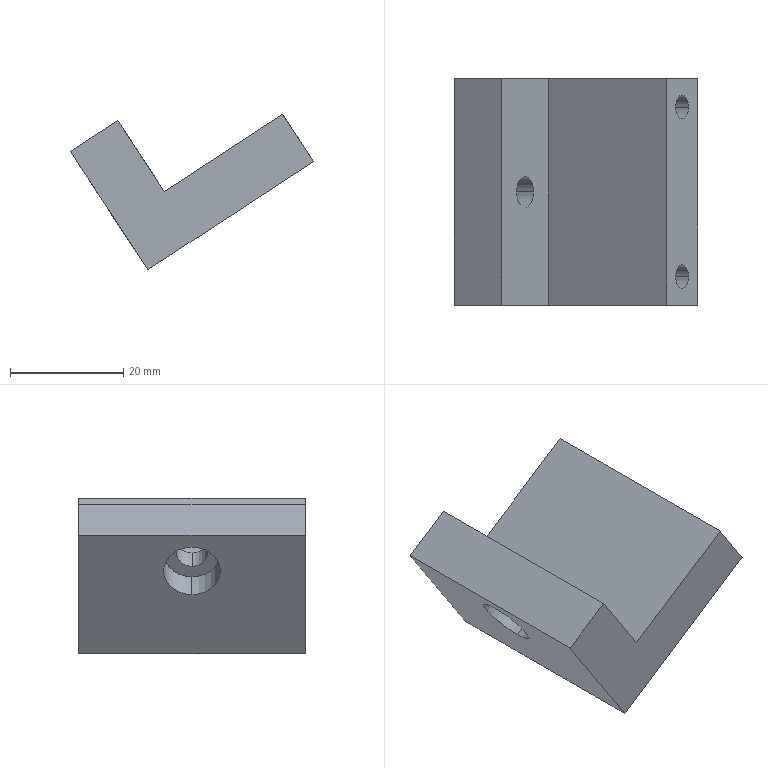Component | SolidWorks | PullSuctionCupMountingPlate-1 | 1 solid | 21 faces | box 42.97 x 40 x 27.52 mm | volume 19095 mm3 | plane 9 | cylinder 8 | cone 4 | commonest cylinder face diameters 4.2 x4 10 x2 5.5 x2
build123d program:
from build123d import *

# Parameters (mm, degrees)
SKETCH1_W                                            = 25
SKETCH1_H                                            = 40
BOSS_EXTRUDE1_DEPTH                                  = 35
SKETCH2_W                                            = 15
SKETCH2_H                                            = 25
CUT_EXTRUDE1_DEPTH                                   = 55.601
M5_TAPPED_HOLE1_D                                    = 4.2
M5_TAPPED_HOLE1_DEPTH                                = 12.4
M5_TAPPED_HOLE1_TIP                                  = 1.262
HOLE_SIZE_ACCORDING_TO_THE_TYPE_OF_HEXAG_D           = 5.5
HOLE_SIZE_ACCORDING_TO_THE_TYPE_OF_HEXAG_CBORE_D     = 10
HOLE_SIZE_ACCORDING_TO_THE_TYPE_OF_HEXAG_CBORE_DEPTH = 5.7


with BuildPart() as part:
    # Sketch1 → Boss-Extrude1 (new body)
    with BuildSketch(Plane.XY):
        Rectangle(SKETCH1_W, SKETCH1_H)
    extrude(amount=BOSS_EXTRUDE1_DEPTH)

    # Sketch2 → Cut-Extrude1 (cut, through all)
    with BuildSketch(Plane(origin=(0, 20, 0), x_dir=(1, 0, 0), z_dir=(0, 1, 0))):
        with Locations((-5, -22.5)):
            Rectangle(SKETCH2_W, SKETCH2_H)
    extrude(amount=-CUT_EXTRUDE1_DEPTH, mode=Mode.SUBTRACT)

    # M5 Tapped Hole1
    with Locations(Plane.XY.offset(35)):
        with Locations((7.5, 15), (7.5, -15)):
            Hole(M5_TAPPED_HOLE1_D / 2, depth=M5_TAPPED_HOLE1_DEPTH)
            with Locations((0, 0, -(M5_TAPPED_HOLE1_DEPTH + M5_TAPPED_HOLE1_TIP / 2))):  # 118° drill point
                Cone(0, M5_TAPPED_HOLE1_D / 2, M5_TAPPED_HOLE1_TIP, mode=Mode.SUBTRACT)

    # Hole Size according to the type of hexag (through all)
    with Locations(Plane(origin=(0, 0, 0), x_dir=(-1, 0, 0), z_dir=(0, 0, -1))):
        with Locations((5, 0)):
            CounterBoreHole(HOLE_SIZE_ACCORDING_TO_THE_TYPE_OF_HEXAG_D / 2, HOLE_SIZE_ACCORDING_TO_THE_TYPE_OF_HEXAG_CBORE_D / 2, HOLE_SIZE_ACCORDING_TO_THE_TYPE_OF_HEXAG_CBORE_DEPTH)


solid = part.part

# Placed as in the assembly
solid = solid.moved(Location((-247.326, -40.454, -152.764), (0, 56.835, 0)))
STEP:
#1=COLOUR_RGB('',0.7922,0.8196,0.9333);
#2=FILL_AREA_STYLE_COLOUR('',#1);
#3=FILL_AREA_STYLE('',(#2));
#4=SURFACE_STYLE_FILL_AREA(#3);
#5=SURFACE_SIDE_STYLE('',(#4));
#6=SURFACE_STYLE_USAGE(.BOTH.,#5);
#7=PRESENTATION_STYLE_ASSIGNMENT((#6));
#8=CARTESIAN_POINT('',(-9.549,-1.593,-5.892));
#9=VERTEX_POINT('',#8);
#10=CARTESIAN_POINT('',(-9.765,-1.593,-5.562));
#11=VERTEX_POINT('',#10);
#12=CARTESIAN_POINT('',(-9.657,-1.593,-5.727));
#13=DIRECTION('',(-0.8371,0.,-0.5471));
#14=DIRECTION('',(-0.5471,-0.,0.8371));
#15=AXIS2_PLACEMENT_3D('',#12,#13,#14);
#16=CIRCLE('',#15,0.1969);
#17=EDGE_CURVE('',#9,#11,#16,.T.);
#18=ORIENTED_EDGE('',*,*,#17,.F.);
#19=CARTESIAN_POINT('',(-9.737,-1.593,-6.014));
#20=VERTEX_POINT('',#19);
#21=CARTESIAN_POINT('',(-9.737,-1.593,-6.014));
#22=DIRECTION('',(-0.8371,0.,-0.5471));
#23=VECTOR('',#22,39.37);
#24=LINE('',#21,#23);
#25=EDGE_CURVE('',#9,#20,#24,.T.);
#26=ORIENTED_EDGE('',*,*,#25,.T.);
#27=CARTESIAN_POINT('',(-9.953,-1.593,-5.685));
#28=VERTEX_POINT('',#27);
#29=CARTESIAN_POINT('',(-9.845,-1.593,-5.85));
#30=DIRECTION('',(-0.8371,0.,-0.5471));
#31=DIRECTION('',(-0.5471,-0.,0.8371));
#32=AXIS2_PLACEMENT_3D('',#29,#30,#31);
#33=CIRCLE('',#32,0.1969);
#34=EDGE_CURVE('',#20,#28,#33,.T.);
#35=ORIENTED_EDGE('',*,*,#34,.T.);
#36=CARTESIAN_POINT('',(-9.953,-1.593,-5.685));
#37=DIRECTION('',(-0.8371,0.,-0.5471));
#38=VECTOR('',#37,39.37);
#39=LINE('',#36,#38);
#40=EDGE_CURVE('',#11,#28,#39,.T.);
#41=ORIENTED_EDGE('',*,*,#40,.F.);
#42=EDGE_LOOP('',(#18,#26,#35,#41));
#43=FACE_OUTER_BOUND('',#42,.T.);
#44=CARTESIAN_POINT('',(-9.845,-1.593,-5.85));
#45=DIRECTION('',(-0.8371,0.,-0.5471));
#46=DIRECTION('',(-0.5471,-0.,0.8371));
#47=AXIS2_PLACEMENT_3D('',#44,#45,#46);
#48=CYLINDRICAL_SURFACE('',#47,0.1969);
#49=ADVANCED_FACE('',(#43),#48,.F.);
#50=CARTESIAN_POINT('',(-9.456,-1.593,-5.725));
#51=VERTEX_POINT('',#50);
#52=CARTESIAN_POINT('',(-9.575,-1.593,-5.544));
#53=VERTEX_POINT('',#52);
#54=CARTESIAN_POINT('',(-9.515,-1.593,-5.634));
#55=DIRECTION('',(-0.8371,0.,-0.5471));
#56=DIRECTION('',(-0.5471,-0.,0.8371));
#57=AXIS2_PLACEMENT_3D('',#54,#55,#56);
#58=CIRCLE('',#57,0.1083);
#59=EDGE_CURVE('',#51,#53,#58,.T.);
#60=ORIENTED_EDGE('',*,*,#59,.F.);
#61=CARTESIAN_POINT('',(-9.598,-1.593,-5.817));
#62=VERTEX_POINT('',#61);
#63=CARTESIAN_POINT('',(-9.786,-1.593,-5.94));
#64=DIRECTION('',(-0.8371,0.,-0.5471));
#65=VECTOR('',#64,39.37);
#66=LINE('',#63,#65);
#67=EDGE_CURVE('',#51,#62,#66,.T.);
#68=ORIENTED_EDGE('',*,*,#67,.T.);
#69=CARTESIAN_POINT('',(-9.716,-1.593,-5.636));
#70=VERTEX_POINT('',#69);
#71=CARTESIAN_POINT('',(-9.657,-1.593,-5.727));
#72=DIRECTION('',(-0.8371,0.,-0.5471));
#73=DIRECTION('',(-0.5471,-0.,0.8371));
#74=AXIS2_PLACEMENT_3D('',#71,#72,#73);
#75=CIRCLE('',#74,0.1083);
#76=EDGE_CURVE('',#62,#70,#75,.T.);
#77=ORIENTED_EDGE('',*,*,#76,.T.);
#78=CARTESIAN_POINT('',(-9.904,-1.593,-5.759));
#79=DIRECTION('',(-0.8371,0.,-0.5471));
#80=VECTOR('',#79,39.37);
#81=LINE('',#78,#80);
#82=EDGE_CURVE('',#53,#70,#81,.T.);
#83=ORIENTED_EDGE('',*,*,#82,.F.);
#84=EDGE_LOOP('',(#60,#68,#77,#83));
#85=FACE_OUTER_BOUND('',#84,.T.);
#86=CARTESIAN_POINT('',(-9.845,-1.593,-5.85));
#87=DIRECTION('',(-0.8371,0.,-0.5471));
#88=DIRECTION('',(-0.5471,-0.,0.8371));
#89=AXIS2_PLACEMENT_3D('',#86,#87,#88);
#90=CYLINDRICAL_SURFACE('',#89,0.1083);
#91=ADVANCED_FACE('',(#85),#90,.F.);
#92=CARTESIAN_POINT('',(-8.876,-1.002,-5.706));
#93=VERTEX_POINT('',#92);
#94=CARTESIAN_POINT('',(-8.786,-1.002,-5.844));
#95=VERTEX_POINT('',#94);
#96=CARTESIAN_POINT('',(-8.831,-1.002,-5.775));
#97=DIRECTION('',(0.8371,-0.,0.5471));
#98=DIRECTION('',(0.5471,0.,-0.8371));
#99=AXIS2_PLACEMENT_3D('',#96,#97,#98);
#100=CIRCLE('',#99,0.08268);
#101=EDGE_CURVE('',#93,#95,#100,.T.);
#102=ORIENTED_EDGE('',*,*,#101,.F.);
#103=CARTESIAN_POINT('',(-8.467,-1.002,-5.438));
#104=VERTEX_POINT('',#103);
#105=CARTESIAN_POINT('',(-8.467,-1.002,-5.438));
#106=DIRECTION('',(0.8371,-0.,0.5471));
#107=VECTOR('',#106,39.37);
#108=LINE('',#105,#107);
#109=EDGE_CURVE('',#93,#104,#108,.T.);
#110=ORIENTED_EDGE('',*,*,#109,.T.);
#111=CARTESIAN_POINT('',(-8.377,-1.002,-5.577));
#112=VERTEX_POINT('',#111);
#113=CARTESIAN_POINT('',(-8.422,-1.002,-5.508));
#114=DIRECTION('',(0.8371,-0.,0.5471));
#115=DIRECTION('',(0.5471,0.,-0.8371));
#116=AXIS2_PLACEMENT_3D('',#113,#114,#115);
#117=CIRCLE('',#116,0.08268);
#118=EDGE_CURVE('',#104,#112,#117,.T.);
#119=ORIENTED_EDGE('',*,*,#118,.T.);
#120=CARTESIAN_POINT('',(-8.377,-1.002,-5.577));
#121=DIRECTION('',(0.8371,-0.,0.5471));
#122=VECTOR('',#121,39.37);
#123=LINE('',#120,#122);
#124=EDGE_CURVE('',#95,#112,#123,.T.);
#125=ORIENTED_EDGE('',*,*,#124,.F.);
#126=EDGE_LOOP('',(#102,#110,#119,#125));
#127=FACE_OUTER_BOUND('',#126,.T.);
#128=CARTESIAN_POINT('',(-8.422,-1.002,-5.508));
#129=DIRECTION('',(0.8371,-0.,0.5471));
#130=DIRECTION('',(0.5471,0.,-0.8371));
#131=AXIS2_PLACEMENT_3D('',#128,#129,#130);
#132=CYLINDRICAL_SURFACE('',#131,0.08268);
#133=ADVANCED_FACE('',(#127),#132,.F.);
#134=CARTESIAN_POINT('',(-8.872,-1.002,-5.802));
#135=VERTEX_POINT('',#134);
#136=CARTESIAN_POINT('',(-8.786,-1.002,-5.844));
#137=DIRECTION('',(0.9001,0.,-0.4358));
#138=VECTOR('',#137,39.37);
#139=LINE('',#136,#138);
#140=EDGE_CURVE('',#135,#95,#139,.T.);
#141=ORIENTED_EDGE('',*,*,#140,.F.);
#142=CARTESIAN_POINT('',(-8.876,-1.002,-5.706));
#143=DIRECTION('',(-0.03778,-0.,0.9993));
#144=VECTOR('',#143,39.37);
#145=LINE('',#142,#144);
#146=EDGE_CURVE('',#135,#93,#145,.T.);
#147=ORIENTED_EDGE('',*,*,#146,.T.);
#148=ORIENTED_EDGE('',*,*,#101,.T.);
#149=EDGE_LOOP('',(#141,#147,#148));
#150=FACE_OUTER_BOUND('',#149,.T.);
#151=CARTESIAN_POINT('',(-8.831,-1.002,-5.775));
#152=DIRECTION('',(0.8371,-0.,0.5471));
#153=DIRECTION('',(0.5471,0.,-0.8371));
#154=AXIS2_PLACEMENT_3D('',#151,#152,#153);
#155=CONICAL_SURFACE('',#154,0.08268,1.03);
#156=ADVANCED_FACE('',(#150),#155,.F.);
#157=CARTESIAN_POINT('',(-8.876,-2.183,-5.706));
#158=VERTEX_POINT('',#157);
#159=CARTESIAN_POINT('',(-8.786,-2.183,-5.844));
#160=VERTEX_POINT('',#159);
#161=CARTESIAN_POINT('',(-8.831,-2.183,-5.775));
#162=DIRECTION('',(0.8371,-0.,0.5471));
#163=DIRECTION('',(0.5471,0.,-0.8371));
#164=AXIS2_PLACEMENT_3D('',#161,#162,#163);
#165=CIRCLE('',#164,0.08268);
#166=EDGE_CURVE('',#158,#160,#165,.T.);
#167=ORIENTED_EDGE('',*,*,#166,.F.);
#168=CARTESIAN_POINT('',(-8.467,-2.183,-5.438));
#169=VERTEX_POINT('',#168);
#170=CARTESIAN_POINT('',(-8.467,-2.183,-5.438));
#171=DIRECTION('',(0.8371,-0.,0.5471));
#172=VECTOR('',#171,39.37);
#173=LINE('',#170,#172);
#174=EDGE_CURVE('',#158,#169,#173,.T.);
#175=ORIENTED_EDGE('',*,*,#174,.T.);
#176=CARTESIAN_POINT('',(-8.377,-2.183,-5.577));
#177=VERTEX_POINT('',#176);
#178=CARTESIAN_POINT('',(-8.422,-2.183,-5.508));
#179=DIRECTION('',(0.8371,-0.,0.5471));
#180=DIRECTION('',(0.5471,0.,-0.8371));
#181=AXIS2_PLACEMENT_3D('',#178,#179,#180);
#182=CIRCLE('',#181,0.08268);
#183=EDGE_CURVE('',#169,#177,#182,.T.);
#184=ORIENTED_EDGE('',*,*,#183,.T.);
#185=CARTESIAN_POINT('',(-8.377,-2.183,-5.577));
#186=DIRECTION('',(0.8371,-0.,0.5471));
#187=VECTOR('',#186,39.37);
#188=LINE('',#185,#187);
#189=EDGE_CURVE('',#160,#177,#188,.T.);
#190=ORIENTED_EDGE('',*,*,#189,.F.);
#191=EDGE_LOOP('',(#167,#175,#184,#190));
#192=FACE_OUTER_BOUND('',#191,.T.);
#193=CARTESIAN_POINT('',(-8.422,-2.183,-5.508));
#194=DIRECTION('',(0.8371,-0.,0.5471));
#195=DIRECTION('',(0.5471,0.,-0.8371));
#196=AXIS2_PLACEMENT_3D('',#193,#194,#195);
#197=CYLINDRICAL_SURFACE('',#196,0.08268);
#198=ADVANCED_FACE('',(#192),#197,.F.);
#199=CARTESIAN_POINT('',(-8.872,-2.183,-5.802));
#200=VERTEX_POINT('',#199);
#201=CARTESIAN_POINT('',(-8.786,-2.183,-5.844));
#202=DIRECTION('',(0.9001,0.,-0.4358));
#203=VECTOR('',#202,39.37);
#204=LINE('',#201,#203);
#205=EDGE_CURVE('',#200,#160,#204,.T.);
#206=ORIENTED_EDGE('',*,*,#205,.F.);
#207=CARTESIAN_POINT('',(-8.876,-2.183,-5.706));
#208=DIRECTION('',(-0.03778,-0.,0.9993));
#209=VECTOR('',#208,39.37);
#210=LINE('',#207,#209);
#211=EDGE_CURVE('',#200,#158,#210,.T.);
#212=ORIENTED_EDGE('',*,*,#211,.T.);
#213=ORIENTED_EDGE('',*,*,#166,.T.);
#214=EDGE_LOOP('',(#206,#212,#213));
#215=FACE_OUTER_BOUND('',#214,.T.);
#216=CARTESIAN_POINT('',(-8.831,-2.183,-5.775));
#217=DIRECTION('',(0.8371,-0.,0.5471));
#218=DIRECTION('',(0.5471,0.,-0.8371));
#219=AXIS2_PLACEMENT_3D('',#216,#217,#218);
#220=CONICAL_SURFACE('',#219,0.08268,1.03);
#221=ADVANCED_FACE('',(#215),#220,.F.);
#222=CARTESIAN_POINT('',(-9.468,-2.38,-6.426));
#223=VERTEX_POINT('',#222);
#224=CARTESIAN_POINT('',(-9.468,-0.8053,-6.426));
#225=VERTEX_POINT('',#224);
#226=CARTESIAN_POINT('',(-9.468,-2.38,-6.426));
#227=DIRECTION('',(-0.,1.,0.));
#228=VECTOR('',#227,39.37);
#229=LINE('',#226,#228);
#230=EDGE_CURVE('',#223,#225,#229,.T.);
#231=ORIENTED_EDGE('',*,*,#230,.T.);
#232=CARTESIAN_POINT('',(-8.315,-0.8053,-5.672));
#233=VERTEX_POINT('',#232);
#234=CARTESIAN_POINT('',(-8.315,-0.8053,-5.672));
#235=DIRECTION('',(-0.8371,0.,-0.5471));
#236=VECTOR('',#235,39.37);
#237=LINE('',#234,#236);
#238=EDGE_CURVE('',#233,#225,#237,.T.);
#239=ORIENTED_EDGE('',*,*,#238,.F.);
#240=CARTESIAN_POINT('',(-8.315,-2.38,-5.672));
#241=VERTEX_POINT('',#240);
#242=CARTESIAN_POINT('',(-8.315,-2.38,-5.672));
#243=DIRECTION('',(-0.,1.,0.));
#244=VECTOR('',#243,39.37);
#245=LINE('',#242,#244);
#246=EDGE_CURVE('',#241,#233,#245,.T.);
#247=ORIENTED_EDGE('',*,*,#246,.F.);
#248=CARTESIAN_POINT('',(-8.315,-2.38,-5.672));
#249=DIRECTION('',(-0.8371,0.,-0.5471));
#250=VECTOR('',#249,39.37);
#251=LINE('',#248,#250);
#252=EDGE_CURVE('',#241,#223,#251,.T.);
#253=ORIENTED_EDGE('',*,*,#252,.T.);
#254=EDGE_LOOP('',(#231,#239,#247,#253));
#255=FACE_OUTER_BOUND('',#254,.T.);
#256=CARTESIAN_POINT('',(-8.315,-2.38,-5.672));
#257=DIRECTION('',(-0.5471,-0.,0.8371));
#258=DIRECTION('',(0.8371,-0.,0.5471));
#259=AXIS2_PLACEMENT_3D('',#256,#257,#258);
#260=PLANE('',#259);
#261=ADVANCED_FACE('',(#255),#260,.F.);
#262=CARTESIAN_POINT('',(-9.677,-0.8053,-5.387));
#263=VERTEX_POINT('',#262);
#264=CARTESIAN_POINT('',(-10.006,-0.8053,-5.602));
#265=VERTEX_POINT('',#264);
#266=CARTESIAN_POINT('',(-8.853,-0.8053,-4.849));
#267=DIRECTION('',(-0.8371,0.,-0.5471));
#268=VECTOR('',#267,39.37);
#269=LINE('',#266,#268);
#270=EDGE_CURVE('',#263,#265,#269,.T.);
#271=ORIENTED_EDGE('',*,*,#270,.F.);
#272=CARTESIAN_POINT('',(-9.354,-0.8053,-5.881));
#273=VERTEX_POINT('',#272);
#274=CARTESIAN_POINT('',(-9.677,-0.8053,-5.387));
#275=DIRECTION('',(-0.5471,-0.,0.8371));
#276=VECTOR('',#275,39.37);
#277=LINE('',#274,#276);
#278=EDGE_CURVE('',#273,#263,#277,.T.);
#279=ORIENTED_EDGE('',*,*,#278,.F.);
#280=CARTESIAN_POINT('',(-8.53,-0.8053,-5.343));
#281=VERTEX_POINT('',#280);
#282=CARTESIAN_POINT('',(-8.53,-0.8053,-5.343));
#283=DIRECTION('',(-0.8371,0.,-0.5471));
#284=VECTOR('',#283,39.37);
#285=LINE('',#282,#284);
#286=EDGE_CURVE('',#281,#273,#285,.T.);
#287=ORIENTED_EDGE('',*,*,#286,.F.);
#288=CARTESIAN_POINT('',(-8.853,-0.8053,-4.849));
#289=DIRECTION('',(-0.5471,-0.,0.8371));
#290=VECTOR('',#289,39.37);
#291=LINE('',#288,#290);
#292=EDGE_CURVE('',#233,#281,#291,.T.);
#293=ORIENTED_EDGE('',*,*,#292,.F.);
#294=ORIENTED_EDGE('',*,*,#238,.T.);
#295=CARTESIAN_POINT('',(-10.006,-0.8053,-5.602));
#296=DIRECTION('',(-0.5471,-0.,0.8371));
#297=VECTOR('',#296,39.37);
#298=LINE('',#295,#297);
#299=EDGE_CURVE('',#225,#265,#298,.T.);
#300=ORIENTED_EDGE('',*,*,#299,.T.);
#301=EDGE_LOOP('',(#271,#279,#287,#293,#294,#300));
#302=FACE_OUTER_BOUND('',#301,.T.);
#303=CARTESIAN_POINT('',(-8.853,-0.8053,-4.849));
#304=DIRECTION('',(0.,-1.,-0.));
#305=DIRECTION('',(-0.8371,0.,-0.5471));
#306=AXIS2_PLACEMENT_3D('',#303,#304,#305);
#307=PLANE('',#306);
#308=ADVANCED_FACE('',(#302),#307,.F.);
#309=CARTESIAN_POINT('',(-9.677,-2.38,-5.387));
#310=VERTEX_POINT('',#309);
#311=CARTESIAN_POINT('',(-10.006,-2.38,-5.602));
#312=VERTEX_POINT('',#311);
#313=CARTESIAN_POINT('',(-8.853,-2.38,-4.849));
#314=DIRECTION('',(-0.8371,0.,-0.5471));
#315=VECTOR('',#314,39.37);
#316=LINE('',#313,#315);
#317=EDGE_CURVE('',#310,#312,#316,.T.);
#318=ORIENTED_EDGE('',*,*,#317,.F.);
#319=CARTESIAN_POINT('',(-9.677,-2.38,-5.387));
#320=DIRECTION('',(-0.,1.,0.));
#321=VECTOR('',#320,39.37);
#322=LINE('',#319,#321);
#323=EDGE_CURVE('',#310,#263,#322,.T.);
#324=ORIENTED_EDGE('',*,*,#323,.T.);
#325=ORIENTED_EDGE('',*,*,#270,.T.);
#326=CARTESIAN_POINT('',(-10.006,-2.38,-5.602));
#327=DIRECTION('',(0.,-1.,-0.));
#328=VECTOR('',#327,39.37);
#329=LINE('',#326,#328);
#330=EDGE_CURVE('',#265,#312,#329,.T.);
#331=ORIENTED_EDGE('',*,*,#330,.T.);
#332=EDGE_LOOP('',(#318,#324,#325,#331));
#333=FACE_OUTER_BOUND('',#332,.T.);
#334=CARTESIAN_POINT('',(-8.853,-2.38,-4.849));
#335=DIRECTION('',(0.5471,0.,-0.8371));
#336=DIRECTION('',(-0.8371,0.,-0.5471));
#337=AXIS2_PLACEMENT_3D('',#334,#335,#336);
#338=PLANE('',#337);
#339=ADVANCED_FACE('',(#333),#338,.F.);
#340=CARTESIAN_POINT('',(-8.53,-2.38,-5.343));
#341=VERTEX_POINT('',#340);
#342=CARTESIAN_POINT('',(-9.354,-2.38,-5.881));
#343=VERTEX_POINT('',#342);
#344=CARTESIAN_POINT('',(-8.53,-2.38,-5.343));
#345=DIRECTION('',(-0.8371,0.,-0.5471));
#346=VECTOR('',#345,39.37);
#347=LINE('',#344,#346);
#348=EDGE_CURVE('',#341,#343,#347,.T.);
#349=ORIENTED_EDGE('',*,*,#348,.T.);
#350=CARTESIAN_POINT('',(-9.677,-2.38,-5.387));
#351=DIRECTION('',(-0.5471,-0.,0.8371));
#352=VECTOR('',#351,39.37);
#353=LINE('',#350,#352);
#354=EDGE_CURVE('',#343,#310,#353,.T.);
#355=ORIENTED_EDGE('',*,*,#354,.T.);
#356=ORIENTED_EDGE('',*,*,#317,.T.);
#357=CARTESIAN_POINT('',(-10.006,-2.38,-5.602));
#358=DIRECTION('',(0.5471,0.,-0.8371));
#359=VECTOR('',#358,39.37);
#360=LINE('',#357,#359);
#361=EDGE_CURVE('',#312,#223,#360,.T.);
#362=ORIENTED_EDGE('',*,*,#361,.T.);
#363=ORIENTED_EDGE('',*,*,#252,.F.);
#364=CARTESIAN_POINT('',(-8.853,-2.38,-4.849));
#365=DIRECTION('',(0.5471,0.,-0.8371));
#366=VECTOR('',#365,39.37);
#367=LINE('',#364,#366);
#368=EDGE_CURVE('',#341,#241,#367,.T.);
#369=ORIENTED_EDGE('',*,*,#368,.F.);
#370=EDGE_LOOP('',(#349,#355,#356,#362,#363,#369));
#371=FACE_OUTER_BOUND('',#370,.T.);
#372=CARTESIAN_POINT('',(-8.853,-2.38,-4.849));
#373=DIRECTION('',(-0.,1.,0.));
#374=DIRECTION('',(0.8371,-0.,0.5471));
#375=AXIS2_PLACEMENT_3D('',#372,#373,#374);
#376=PLANE('',#375);
#377=ADVANCED_FACE('',(#371),#376,.F.);
#378=CARTESIAN_POINT('',(-8.422,-1.002,-5.508));
#379=DIRECTION('',(0.8371,-0.,0.5471));
#380=DIRECTION('',(0.5471,0.,-0.8371));
#381=AXIS2_PLACEMENT_3D('',#378,#379,#380);
#382=CIRCLE('',#381,0.08268);
#383=EDGE_CURVE('',#112,#104,#382,.T.);
#384=ORIENTED_EDGE('',*,*,#383,.F.);
#385=ORIENTED_EDGE('',*,*,#118,.F.);
#386=EDGE_LOOP('',(#384,#385));
#387=FACE_BOUND('',#386,.T.);
#388=CARTESIAN_POINT('',(-8.422,-2.183,-5.508));
#389=DIRECTION('',(0.8371,-0.,0.5471));
#390=DIRECTION('',(0.5471,0.,-0.8371));
#391=AXIS2_PLACEMENT_3D('',#388,#389,#390);
#392=CIRCLE('',#391,0.08268);
#393=EDGE_CURVE('',#177,#169,#392,.T.);
#394=ORIENTED_EDGE('',*,*,#393,.F.);
#395=ORIENTED_EDGE('',*,*,#183,.F.);
#396=EDGE_LOOP('',(#394,#395));
#397=FACE_BOUND('',#396,.T.);
#398=ORIENTED_EDGE('',*,*,#292,.T.);
#399=CARTESIAN_POINT('',(-8.53,-2.38,-5.343));
#400=DIRECTION('',(-0.,1.,0.));
#401=VECTOR('',#400,39.37);
#402=LINE('',#399,#401);
#403=EDGE_CURVE('',#341,#281,#402,.T.);
#404=ORIENTED_EDGE('',*,*,#403,.F.);
#405=ORIENTED_EDGE('',*,*,#368,.T.);
#406=ORIENTED_EDGE('',*,*,#246,.T.);
#407=EDGE_LOOP('',(#398,#404,#405,#406));
#408=FACE_OUTER_BOUND('',#407,.T.);
#409=CARTESIAN_POINT('',(-8.584,-1.593,-5.261));
#410=DIRECTION('',(-0.8371,0.,-0.5471));
#411=DIRECTION('',(-0.5471,-0.,0.8371));
#412=AXIS2_PLACEMENT_3D('',#409,#410,#411);
#413=PLANE('',#412);
#414=ADVANCED_FACE('',(#387,#397,#408),#413,.F.);
#415=CARTESIAN_POINT('',(-9.845,-1.593,-5.85));
#416=DIRECTION('',(-0.8371,0.,-0.5471));
#417=DIRECTION('',(-0.5471,-0.,0.8371));
#418=AXIS2_PLACEMENT_3D('',#415,#416,#417);
#419=CIRCLE('',#418,0.1969);
#420=EDGE_CURVE('',#28,#20,#419,.T.);
#421=ORIENTED_EDGE('',*,*,#420,.F.);
#422=ORIENTED_EDGE('',*,*,#34,.F.);
#423=EDGE_LOOP('',(#421,#422));
#424=FACE_BOUND('',#423,.T.);
#425=ORIENTED_EDGE('',*,*,#230,.F.);
#426=ORIENTED_EDGE('',*,*,#361,.F.);
#427=ORIENTED_EDGE('',*,*,#330,.F.);
#428=ORIENTED_EDGE('',*,*,#299,.F.);
#429=EDGE_LOOP('',(#425,#426,#427,#428));
#430=FACE_OUTER_BOUND('',#429,.T.);
#431=CARTESIAN_POINT('',(-9.737,-1.593,-6.014));
#432=DIRECTION('',(-0.8371,0.,-0.5471));
#433=DIRECTION('',(-0.5471,-0.,0.8371));
#434=AXIS2_PLACEMENT_3D('',#431,#432,#433);
#435=PLANE('',#434);
#436=ADVANCED_FACE('',(#424,#430),#435,.T.);
#437=CARTESIAN_POINT('',(-9.515,-1.593,-5.634));
#438=DIRECTION('',(-0.8371,0.,-0.5471));
#439=DIRECTION('',(-0.5471,-0.,0.8371));
#440=AXIS2_PLACEMENT_3D('',#437,#438,#439);
#441=CIRCLE('',#440,0.1083);
#442=EDGE_CURVE('',#53,#51,#441,.T.);
#443=ORIENTED_EDGE('',*,*,#442,.T.);
#444=ORIENTED_EDGE('',*,*,#59,.T.);
#445=EDGE_LOOP('',(#443,#444));
#446=FACE_BOUND('',#445,.T.);
#447=ORIENTED_EDGE('',*,*,#278,.T.);
#448=ORIENTED_EDGE('',*,*,#323,.F.);
#449=ORIENTED_EDGE('',*,*,#354,.F.);
#450=CARTESIAN_POINT('',(-9.354,-2.38,-5.881));
#451=DIRECTION('',(-0.,1.,0.));
#452=VECTOR('',#451,39.37);
#453=LINE('',#450,#452);
#454=EDGE_CURVE('',#343,#273,#453,.T.);
#455=ORIENTED_EDGE('',*,*,#454,.T.);
#456=EDGE_LOOP('',(#447,#448,#449,#455));
#457=FACE_OUTER_BOUND('',#456,.T.);
#458=CARTESIAN_POINT('',(-9.677,-2.38,-5.387));
#459=DIRECTION('',(-0.8371,0.,-0.5471));
#460=DIRECTION('',(-0.5471,-0.,0.8371));
#461=AXIS2_PLACEMENT_3D('',#458,#459,#460);
#462=PLANE('',#461);
#463=ADVANCED_FACE('',(#446,#457),#462,.F.);
#464=ORIENTED_EDGE('',*,*,#286,.T.);
#465=ORIENTED_EDGE('',*,*,#454,.F.);
#466=ORIENTED_EDGE('',*,*,#348,.F.);
#467=ORIENTED_EDGE('',*,*,#403,.T.);
#468=EDGE_LOOP('',(#464,#465,#466,#467));
#469=FACE_OUTER_BOUND('',#468,.T.);
#470=CARTESIAN_POINT('',(-8.53,-2.38,-5.343));
#471=DIRECTION('',(0.5471,0.,-0.8371));
#472=DIRECTION('',(-0.8371,0.,-0.5471));
#473=AXIS2_PLACEMENT_3D('',#470,#471,#472);
#474=PLANE('',#473);
#475=ADVANCED_FACE('',(#469),#474,.F.);
#476=ORIENTED_EDGE('',*,*,#211,.F.);
#477=ORIENTED_EDGE('',*,*,#205,.T.);
#478=CARTESIAN_POINT('',(-8.831,-2.183,-5.775));
#479=DIRECTION('',(0.8371,-0.,0.5471));
#480=DIRECTION('',(0.5471,0.,-0.8371));
#481=AXIS2_PLACEMENT_3D('',#478,#479,#480);
#482=CIRCLE('',#481,0.08268);
#483=EDGE_CURVE('',#160,#158,#482,.T.);
#484=ORIENTED_EDGE('',*,*,#483,.T.);
#485=EDGE_LOOP('',(#476,#477,#484));
#486=FACE_OUTER_BOUND('',#485,.T.);
#487=CARTESIAN_POINT('',(-8.831,-2.183,-5.775));
#488=DIRECTION('',(0.8371,-0.,0.5471));
#489=DIRECTION('',(0.5471,0.,-0.8371));
#490=AXIS2_PLACEMENT_3D('',#487,#488,#489);
#491=CONICAL_SURFACE('',#490,0.08268,1.03);
#492=ADVANCED_FACE('',(#486),#491,.F.);
#493=ORIENTED_EDGE('',*,*,#174,.F.);
#494=ORIENTED_EDGE('',*,*,#483,.F.);
#495=ORIENTED_EDGE('',*,*,#189,.T.);
#496=ORIENTED_EDGE('',*,*,#393,.T.);
#497=EDGE_LOOP('',(#493,#494,#495,#496));
#498=FACE_OUTER_BOUND('',#497,.T.);
#499=CARTESIAN_POINT('',(-8.422,-2.183,-5.508));
#500=DIRECTION('',(0.8371,-0.,0.5471));
#501=DIRECTION('',(0.5471,0.,-0.8371));
#502=AXIS2_PLACEMENT_3D('',#499,#500,#501);
#503=CYLINDRICAL_SURFACE('',#502,0.08268);
#504=ADVANCED_FACE('',(#498),#503,.F.);
#505=ORIENTED_EDGE('',*,*,#146,.F.);
#506=ORIENTED_EDGE('',*,*,#140,.T.);
#507=CARTESIAN_POINT('',(-8.831,-1.002,-5.775));
#508=DIRECTION('',(0.8371,-0.,0.5471));
#509=DIRECTION('',(0.5471,0.,-0.8371));
#510=AXIS2_PLACEMENT_3D('',#507,#508,#509);
#511=CIRCLE('',#510,0.08268);
#512=EDGE_CURVE('',#95,#93,#511,.T.);
#513=ORIENTED_EDGE('',*,*,#512,.T.);
#514=EDGE_LOOP('',(#505,#506,#513));
#515=FACE_OUTER_BOUND('',#514,.T.);
#516=CARTESIAN_POINT('',(-8.831,-1.002,-5.775));
#517=DIRECTION('',(0.8371,-0.,0.5471));
#518=DIRECTION('',(0.5471,0.,-0.8371));
#519=AXIS2_PLACEMENT_3D('',#516,#517,#518);
#520=CONICAL_SURFACE('',#519,0.08268,1.03);
#521=ADVANCED_FACE('',(#515),#520,.F.);
#522=ORIENTED_EDGE('',*,*,#109,.F.);
#523=ORIENTED_EDGE('',*,*,#512,.F.);
#524=ORIENTED_EDGE('',*,*,#124,.T.);
#525=ORIENTED_EDGE('',*,*,#383,.T.);
#526=EDGE_LOOP('',(#522,#523,#524,#525));
#527=FACE_OUTER_BOUND('',#526,.T.);
#528=CARTESIAN_POINT('',(-8.422,-1.002,-5.508));
#529=DIRECTION('',(0.8371,-0.,0.5471));
#530=DIRECTION('',(0.5471,0.,-0.8371));
#531=AXIS2_PLACEMENT_3D('',#528,#529,#530);
#532=CYLINDRICAL_SURFACE('',#531,0.08268);
#533=ADVANCED_FACE('',(#527),#532,.F.);
#534=ORIENTED_EDGE('',*,*,#67,.F.);
#535=ORIENTED_EDGE('',*,*,#442,.F.);
#536=ORIENTED_EDGE('',*,*,#82,.T.);
#537=CARTESIAN_POINT('',(-9.657,-1.593,-5.727));
#538=DIRECTION('',(-0.8371,0.,-0.5471));
#539=DIRECTION('',(-0.5471,-0.,0.8371));
#540=AXIS2_PLACEMENT_3D('',#537,#538,#539);
#541=CIRCLE('',#540,0.1083);
#542=EDGE_CURVE('',#70,#62,#541,.T.);
#543=ORIENTED_EDGE('',*,*,#542,.T.);
#544=EDGE_LOOP('',(#534,#535,#536,#543));
#545=FACE_OUTER_BOUND('',#544,.T.);
#546=CARTESIAN_POINT('',(-9.845,-1.593,-5.85));
#547=DIRECTION('',(-0.8371,0.,-0.5471));
#548=DIRECTION('',(-0.5471,-0.,0.8371));
#549=AXIS2_PLACEMENT_3D('',#546,#547,#548);
#550=CYLINDRICAL_SURFACE('',#549,0.1083);
#551=ADVANCED_FACE('',(#545),#550,.F.);
#552=ORIENTED_EDGE('',*,*,#542,.F.);
#553=ORIENTED_EDGE('',*,*,#76,.F.);
#554=EDGE_LOOP('',(#552,#553));
#555=FACE_BOUND('',#554,.T.);
#556=CARTESIAN_POINT('',(-9.657,-1.593,-5.727));
#557=DIRECTION('',(-0.8371,0.,-0.5471));
#558=DIRECTION('',(-0.5471,-0.,0.8371));
#559=AXIS2_PLACEMENT_3D('',#556,#557,#558);
#560=CIRCLE('',#559,0.1969);
#561=EDGE_CURVE('',#11,#9,#560,.T.);
#562=ORIENTED_EDGE('',*,*,#561,.T.);
#563=ORIENTED_EDGE('',*,*,#17,.T.);
#564=EDGE_LOOP('',(#562,#563));
#565=FACE_OUTER_BOUND('',#564,.T.);
#566=CARTESIAN_POINT('',(-9.598,-1.593,-5.817));
#567=DIRECTION('',(0.8371,-0.,0.5471));
#568=DIRECTION('',(0.5471,0.,-0.8371));
#569=AXIS2_PLACEMENT_3D('',#566,#567,#568);
#570=PLANE('',#569);
#571=ADVANCED_FACE('',(#555,#565),#570,.F.);
#572=ORIENTED_EDGE('',*,*,#25,.F.);
#573=ORIENTED_EDGE('',*,*,#561,.F.);
#574=ORIENTED_EDGE('',*,*,#40,.T.);
#575=ORIENTED_EDGE('',*,*,#420,.T.);
#576=EDGE_LOOP('',(#572,#573,#574,#575));
#577=FACE_OUTER_BOUND('',#576,.T.);
#578=CARTESIAN_POINT('',(-9.845,-1.593,-5.85));
#579=DIRECTION('',(-0.8371,0.,-0.5471));
#580=DIRECTION('',(-0.5471,-0.,0.8371));
#581=AXIS2_PLACEMENT_3D('',#578,#579,#580);
#582=CYLINDRICAL_SURFACE('',#581,0.1969);
#583=ADVANCED_FACE('',(#577),#582,.F.);
#584=CLOSED_SHELL('',(#49,#91,#133,#156,#198,#221,#261,#308,#339,#377,#414,#436,#463,#475,#492,#504,#521,#533,#551,#571,#583));
#585=MANIFOLD_SOLID_BREP('',#584);
#586=STYLED_ITEM('',(#7),#585);
#587=PRESENTATION_LAYER_ASSIGNMENT('','',(#586));
#588=(LENGTH_UNIT()NAMED_UNIT(*)SI_UNIT($,.METRE.));
#589=LENGTH_MEASURE_WITH_UNIT(LENGTH_MEASURE(0.0254),#588);
#590=DIMENSIONAL_EXPONENTS(1.,0.,0.,0.,0.,0.,0.);
#591=(CONVERSION_BASED_UNIT('',#589)LENGTH_UNIT()NAMED_UNIT(#590));
#592=UNCERTAINTY_MEASURE_WITH_UNIT(LENGTH_MEASURE(0.00001),#591,'','');
#593=(NAMED_UNIT(*)PLANE_ANGLE_UNIT()SI_UNIT($,.RADIAN.));
#594=(NAMED_UNIT(*)SI_UNIT($,.STERADIAN.)SOLID_ANGLE_UNIT());
#595=(GEOMETRIC_REPRESENTATION_CONTEXT(3)GLOBAL_UNCERTAINTY_ASSIGNED_CONTEXT((#592))GLOBAL_UNIT_ASSIGNED_CONTEXT((#591,#593,#594))REPRESENTATION_CONTEXT('',''));
#596=MECHANICAL_DESIGN_GEOMETRIC_PRESENTATION_REPRESENTATION('',(#586),#595);
#597=CARTESIAN_POINT('',(0.,0.,0.));
#598=DIRECTION('',(0.,0.,1.));
#599=DIRECTION('',(1.,0.,0.));
#600=AXIS2_PLACEMENT_3D('',#597,#598,#599);
#601=(LENGTH_UNIT()NAMED_UNIT(*)SI_UNIT($,.METRE.));
#602=LENGTH_MEASURE_WITH_UNIT(LENGTH_MEASURE(0.0254),#601);
#603=DIMENSIONAL_EXPONENTS(1.,0.,0.,0.,0.,0.,0.);
#604=(CONVERSION_BASED_UNIT('',#602)LENGTH_UNIT()NAMED_UNIT(#603));
#605=UNCERTAINTY_MEASURE_WITH_UNIT(LENGTH_MEASURE(0.00001),#604,'','');
#606=(NAMED_UNIT(*)PLANE_ANGLE_UNIT()SI_UNIT($,.RADIAN.));
#607=(NAMED_UNIT(*)SI_UNIT($,.STERADIAN.)SOLID_ANGLE_UNIT());
#608=(GEOMETRIC_REPRESENTATION_CONTEXT(3)GLOBAL_UNCERTAINTY_ASSIGNED_CONTEXT((#605))GLOBAL_UNIT_ASSIGNED_CONTEXT((#604,#606,#607))REPRESENTATION_CONTEXT('',''));
#609=ADVANCED_BREP_SHAPE_REPRESENTATION('',(#585,#600),#608);